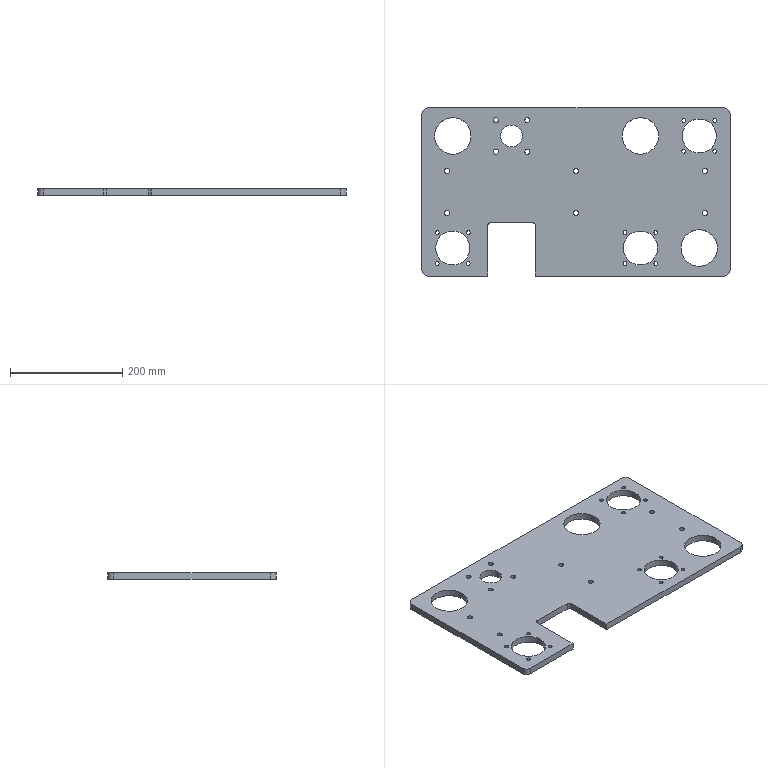Component | SolidWorks | CylinderFixingPlate-1 | 1 solid | 74 faces | box 550 x 300 x 12 mm | volume 1630332 mm3 | cylinder 64 | plane 10 | commonest cylinder face diameters 6.8 x24 9 x20 65 x6 61 x6 20 x4 39 x2 10 x2 | material 6063
build123d program:
from build123d import *

# Parameters (mm, degrees)
SKETCH1_W                    = 550
SKETCH1_H                    = 300
BOSS_EXTRUDE1_DEPTH          = 12
FILLET1_R                    = 10
SKETCH10_R                   = 30.5
SKETCH10_R_2                 = 32.5
SKETCH10_R_3                 = 19.5
SKETCH10_R_4                 = 4.5
CUT_EXTRUDE8_DEPTH           = 314.479
SKETCH11_W                   = 85
SKETCH11_H                   = 95
CUT_EXTRUDE9_DEPTH           = 314.479
FILLET2_R                    = 5
M8_TAPPED_HOLE1_D            = 6.8
M8_TAPPED_HOLE1_DEPTH        = 19.75
M8_TAPPED_HOLE1_TIP          = 2.043
F_9_0_9_DIAMETER_HOLE1_D     = 9
F_9_0_9_DIAMETER_HOLE1_DEPTH = 100
F_9_0_9_DIAMETER_HOLE1_TIP   = 2.598


with BuildPart() as part:
    # Sketch1 → Boss-Extrude1 (new body)
    with BuildSketch(Plane.XY):
        Rectangle(SKETCH1_W, SKETCH1_H)
    extrude(amount=BOSS_EXTRUDE1_DEPTH)

    # Fillet1
    fillet1_edges = [part.edges().sort_by_distance(p)[0] for p in [
        (275, -150, 6),
        (-275, -150, 6),
        (-275, 150, 6),
        (275, 150, 6),
    ]]
    fillet(fillet1_edges, radius=FILLET1_R)

    # Sketch10 → Cut-Extrude8 (cut, through all)
    with BuildSketch(Plane.XY.offset(12)):
        with Locations((-220, -100)):
            Circle(SKETCH10_R)
        with Locations((220, 100)):
            Circle(SKETCH10_R)
        with Locations((115, -100)):
            Circle(SKETCH10_R)
        with Locations((115, 100)):
            Circle(SKETCH10_R_2)
        with Locations((220, -100)):
            Circle(SKETCH10_R_2)
        with Locations((-220, 100)):
            Circle(SKETCH10_R_2)
        with Locations((-115, 100)):
            Circle(SKETCH10_R_3)
        with Locations((-143, 128)):
            Circle(SKETCH10_R_4)
        with Locations((-87, 128)):
            Circle(SKETCH10_R_4)
        with Locations((-87, 72)):
            Circle(SKETCH10_R_4)
        with Locations((-143, 72)):
            Circle(SKETCH10_R_4)
    extrude(amount=-CUT_EXTRUDE8_DEPTH, mode=Mode.SUBTRACT)

    # Sketch11 → Cut-Extrude9 (cut, through all)
    with BuildSketch(Plane.XY.offset(12)):
        with Locations((-115, -102.5)):
            Rectangle(SKETCH11_W, SKETCH11_H)
    extrude(amount=-CUT_EXTRUDE9_DEPTH, mode=Mode.SUBTRACT)

    # Fillet2
    fillet2_edges = [part.edges().sort_by_distance(p)[0] for p in [
        (-72.5, -55, 6),
        (-157.5, -55, 6),
    ]]
    fillet(fillet2_edges, radius=FILLET2_R)

    # M8 Tapped Hole1
    with Locations(Plane(origin=(-192.423, -72.423, 12), x_dir=(1, 0, 0), z_dir=(0, 0, 1))):
        with Locations((0, 0), (-55.154, 0), (-55.154, -55.154), (0, -55.154), (384.846, 200), (440, 200), (440, 144.846), (384.846, 144.846), (335, 0), (279.846, 0), (279.846, -55.154), (335, -55.154)):
            Hole(M8_TAPPED_HOLE1_D / 2, depth=M8_TAPPED_HOLE1_DEPTH)
            with Locations((0, 0, -(M8_TAPPED_HOLE1_DEPTH + M8_TAPPED_HOLE1_TIP / 2))):  # 118° drill point
                Cone(0, M8_TAPPED_HOLE1_D / 2, M8_TAPPED_HOLE1_TIP, mode=Mode.SUBTRACT)

    # 9.0 _9_ Diameter Hole1
    with Locations(Plane(origin=(-230, 37.5, 12), x_dir=(1, 0, 0), z_dir=(0, 0, 1))):
        with Locations((0, 0), (0, -75), (230, -75), (230, 0), (460, 0), (460, -75)):
            Hole(F_9_0_9_DIAMETER_HOLE1_D / 2, depth=F_9_0_9_DIAMETER_HOLE1_DEPTH)
            with Locations((0, 0, -(F_9_0_9_DIAMETER_HOLE1_DEPTH + F_9_0_9_DIAMETER_HOLE1_TIP / 2))):  # 120° drill point
                Cone(0, F_9_0_9_DIAMETER_HOLE1_D / 2, F_9_0_9_DIAMETER_HOLE1_TIP, mode=Mode.SUBTRACT)


solid = part.part

# Placed as in the assembly
solid = solid.moved(Location((1.785, 3.083, -458.966), (0, 0, 0)))